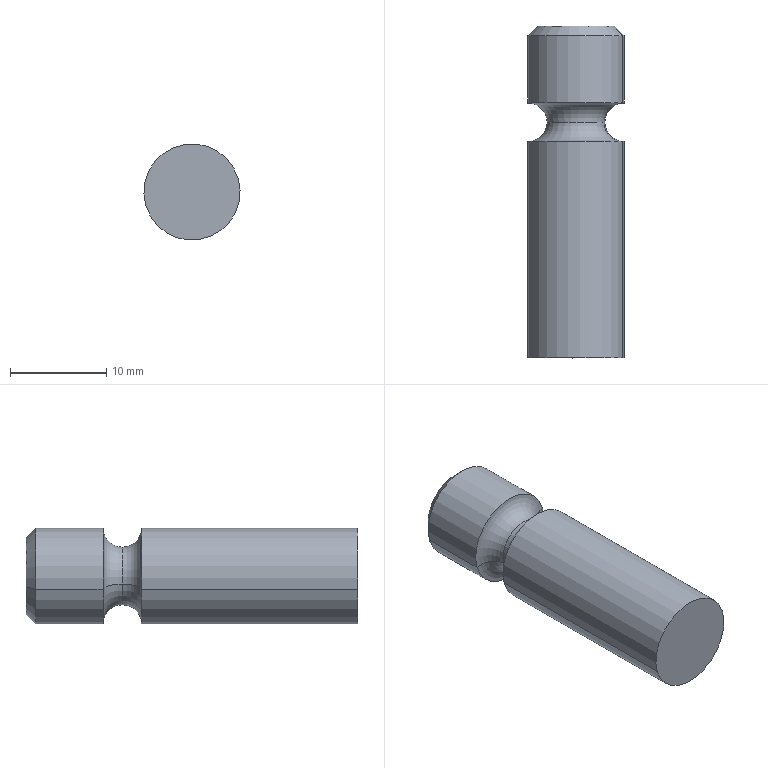Component | SolidWorks | 32-1 | 1 solid | 12 faces | box 10 x 34.5 x 10 mm | volume 2531 mm3 | torus 4 | cylinder 4 | cone 2 | plane 2 | commonest cylinder face diameters 10 x4
build123d program:
from build123d import *

# Parameters (mm, degrees)
SKETCH1_2_R             = 5
BOSS_EXTRUDE1_DEPTH     = 48
CHAMFER1_SIZE           = 1
CHAMFER2_SIZE           = 1
SKETCH3_R               = 2
CUT_EXTRUDE1_DEPTH      = 13.5
CUT_EXTRUDE1_DEPTH_BACK = 13.5
SKETCH1_R               = 6


with BuildPart() as part:
    # Sketch1_2 → Boss-Extrude1 (new body)
    with BuildSketch(Plane.XY):
        Circle(SKETCH1_2_R)
    extrude(amount=BOSS_EXTRUDE1_DEPTH)

    # Chamfer1
    chamfer1_edges = [part.edges().sort_by_distance(p)[0] for p in [
        (-5, 0, 0),
    ]]
    chamfer(chamfer1_edges, length=CHAMFER1_SIZE)

    # Chamfer2
    chamfer2_edges = [part.edges().sort_by_distance(p)[0] for p in [
        (-5, 0, 48),
    ]]
    chamfer(chamfer2_edges, length=CHAMFER2_SIZE)

    # Sketch3 → Cut-Revolve1 (revolve, cut)
    with BuildSketch(Plane(origin=(0, 0, 0), x_dir=(1, 0, 0), z_dir=(0, 1, 0))):
        with Locations((5, -38)):
            Circle(SKETCH3_R)
    revolve(axis=Axis((0, 0, 48), (0, 0, -1)), mode=Mode.SUBTRACT)

    # Sketch1 → Cut-Extrude1 (cut, two sides: drawn at the far end of the back side and taken through both)
    with BuildSketch(Plane.XY.offset(-CUT_EXTRUDE1_DEPTH_BACK)):
        Circle(SKETCH1_R)
    extrude(amount=CUT_EXTRUDE1_DEPTH + CUT_EXTRUDE1_DEPTH_BACK, mode=Mode.SUBTRACT)


solid = part.part

# Placed as in the assembly
solid = solid.moved(Location((17.957, 384.991, 382.093), (-90, 0, 0)))
STEP:
#1=CARTESIAN_POINT('',(0.518,16.732,14.988));
#2=VERTEX_POINT('',#1);
#3=CARTESIAN_POINT('',(0.5936,16.653,15.01));
#4=VERTEX_POINT('',#3);
#5=CARTESIAN_POINT('',(0.518,16.653,14.988));
#6=DIRECTION('',(0.2793,0.,-0.9602));
#7=DIRECTION('',(-0.9602,0.,-0.2793));
#8=AXIS2_PLACEMENT_3D('',#5,#6,#7);
#9=CIRCLE('',#8,0.07874);
#10=EDGE_CURVE('',#2,#4,#9,.T.);
#11=ORIENTED_EDGE('',*,*,#10,.T.);
#12=CARTESIAN_POINT('',(0.8204,16.653,15.076));
#13=VERTEX_POINT('',#12);
#14=CARTESIAN_POINT('',(0.707,16.653,15.043));
#15=DIRECTION('',(-0.,1.,0.));
#16=DIRECTION('',(-1.,0.,0.));
#17=AXIS2_PLACEMENT_3D('',#14,#15,#16);
#18=CIRCLE('',#17,0.1181);
#19=EDGE_CURVE('',#4,#13,#18,.T.);
#20=ORIENTED_EDGE('',*,*,#19,.T.);
#21=CARTESIAN_POINT('',(0.896,16.732,15.098));
#22=VERTEX_POINT('',#21);
#23=CARTESIAN_POINT('',(0.896,16.653,15.098));
#24=DIRECTION('',(-0.2793,-0.,0.9602));
#25=DIRECTION('',(0.9602,0.,0.2793));
#26=AXIS2_PLACEMENT_3D('',#23,#24,#25);
#27=CIRCLE('',#26,0.07874);
#28=EDGE_CURVE('',#22,#13,#27,.T.);
#29=ORIENTED_EDGE('',*,*,#28,.F.);
#30=CARTESIAN_POINT('',(0.707,16.732,15.043));
#31=DIRECTION('',(-0.,1.,0.));
#32=DIRECTION('',(0.9602,0.,0.2793));
#33=AXIS2_PLACEMENT_3D('',#30,#31,#32);
#34=CIRCLE('',#33,0.1969);
#35=EDGE_CURVE('',#2,#22,#34,.T.);
#36=ORIENTED_EDGE('',*,*,#35,.F.);
#37=EDGE_LOOP('',(#11,#20,#29,#36));
#38=FACE_OUTER_BOUND('',#37,.T.);
#39=CARTESIAN_POINT('',(0.707,16.653,15.043));
#40=DIRECTION('',(-0.,1.,0.));
#41=DIRECTION('',(-0.9602,-0.,-0.2793));
#42=AXIS2_PLACEMENT_3D('',#39,#40,#41);
#43=TOROIDAL_SURFACE('',#42,0.1969,0.07874);
#44=ADVANCED_FACE('',(#38),#43,.F.);
#45=ORIENTED_EDGE('',*,*,#28,.T.);
#46=CARTESIAN_POINT('',(0.707,16.653,15.043));
#47=DIRECTION('',(-0.,1.,0.));
#48=DIRECTION('',(-1.,0.,0.));
#49=AXIS2_PLACEMENT_3D('',#46,#47,#48);
#50=CIRCLE('',#49,0.1181);
#51=EDGE_CURVE('',#13,#4,#50,.T.);
#52=ORIENTED_EDGE('',*,*,#51,.T.);
#53=ORIENTED_EDGE('',*,*,#10,.F.);
#54=CARTESIAN_POINT('',(0.707,16.732,15.043));
#55=DIRECTION('',(-0.,1.,0.));
#56=DIRECTION('',(0.9602,0.,0.2793));
#57=AXIS2_PLACEMENT_3D('',#54,#55,#56);
#58=CIRCLE('',#57,0.1969);
#59=EDGE_CURVE('',#22,#2,#58,.T.);
#60=ORIENTED_EDGE('',*,*,#59,.F.);
#61=EDGE_LOOP('',(#45,#52,#53,#60));
#62=FACE_OUTER_BOUND('',#61,.T.);
#63=CARTESIAN_POINT('',(0.707,16.653,15.043));
#64=DIRECTION('',(-0.,1.,0.));
#65=DIRECTION('',(-0.9602,-0.,-0.2793));
#66=AXIS2_PLACEMENT_3D('',#63,#64,#65);
#67=TOROIDAL_SURFACE('',#66,0.1969,0.07874);
#68=ADVANCED_FACE('',(#62),#67,.F.);
#69=CARTESIAN_POINT('',(0.896,16.574,15.098));
#70=VERTEX_POINT('',#69);
#71=CARTESIAN_POINT('',(0.518,16.574,14.988));
#72=VERTEX_POINT('',#71);
#73=CARTESIAN_POINT('',(0.707,16.574,15.043));
#74=DIRECTION('',(0.,-1.,-0.));
#75=DIRECTION('',(-0.9602,0.,-0.2793));
#76=AXIS2_PLACEMENT_3D('',#73,#74,#75);
#77=CIRCLE('',#76,0.1969);
#78=EDGE_CURVE('',#70,#72,#77,.T.);
#79=ORIENTED_EDGE('',*,*,#78,.T.);
#80=CARTESIAN_POINT('',(0.518,15.689,14.988));
#81=VERTEX_POINT('',#80);
#82=CARTESIAN_POINT('',(0.518,17.047,14.988));
#83=DIRECTION('',(0.,-1.,-0.));
#84=VECTOR('',#83,39.37);
#85=LINE('',#82,#84);
#86=EDGE_CURVE('',#72,#81,#85,.T.);
#87=ORIENTED_EDGE('',*,*,#86,.T.);
#88=CARTESIAN_POINT('',(0.896,15.689,15.098));
#89=VERTEX_POINT('',#88);
#90=CARTESIAN_POINT('',(0.707,15.689,15.043));
#91=DIRECTION('',(-0.,1.,0.));
#92=DIRECTION('',(-0.9602,0.,-0.2793));
#93=AXIS2_PLACEMENT_3D('',#90,#91,#92);
#94=CIRCLE('',#93,0.1969);
#95=EDGE_CURVE('',#81,#89,#94,.T.);
#96=ORIENTED_EDGE('',*,*,#95,.T.);
#97=CARTESIAN_POINT('',(0.896,17.047,15.098));
#98=DIRECTION('',(0.,-1.,-0.));
#99=VECTOR('',#98,39.37);
#100=LINE('',#97,#99);
#101=EDGE_CURVE('',#70,#89,#100,.T.);
#102=ORIENTED_EDGE('',*,*,#101,.F.);
#103=EDGE_LOOP('',(#79,#87,#96,#102));
#104=FACE_OUTER_BOUND('',#103,.T.);
#105=CARTESIAN_POINT('',(0.707,17.047,15.043));
#106=DIRECTION('',(0.,-1.,-0.));
#107=DIRECTION('',(0.9602,0.,0.2793));
#108=AXIS2_PLACEMENT_3D('',#105,#106,#107);
#109=CYLINDRICAL_SURFACE('',#108,0.1969);
#110=ADVANCED_FACE('',(#104),#109,.T.);
#111=ORIENTED_EDGE('',*,*,#51,.F.);
#112=CARTESIAN_POINT('',(0.896,16.653,15.098));
#113=DIRECTION('',(-0.2793,-0.,0.9602));
#114=DIRECTION('',(0.9602,0.,0.2793));
#115=AXIS2_PLACEMENT_3D('',#112,#113,#114);
#116=CIRCLE('',#115,0.07874);
#117=EDGE_CURVE('',#13,#70,#116,.T.);
#118=ORIENTED_EDGE('',*,*,#117,.T.);
#119=CARTESIAN_POINT('',(0.707,16.574,15.043));
#120=DIRECTION('',(0.,-1.,-0.));
#121=DIRECTION('',(-0.9602,0.,-0.2793));
#122=AXIS2_PLACEMENT_3D('',#119,#120,#121);
#123=CIRCLE('',#122,0.1969);
#124=EDGE_CURVE('',#72,#70,#123,.T.);
#125=ORIENTED_EDGE('',*,*,#124,.F.);
#126=CARTESIAN_POINT('',(0.518,16.653,14.988));
#127=DIRECTION('',(0.2793,0.,-0.9602));
#128=DIRECTION('',(-0.9602,0.,-0.2793));
#129=AXIS2_PLACEMENT_3D('',#126,#127,#128);
#130=CIRCLE('',#129,0.07874);
#131=EDGE_CURVE('',#4,#72,#130,.T.);
#132=ORIENTED_EDGE('',*,*,#131,.F.);
#133=EDGE_LOOP('',(#111,#118,#125,#132));
#134=FACE_OUTER_BOUND('',#133,.T.);
#135=CARTESIAN_POINT('',(0.707,16.653,15.043));
#136=DIRECTION('',(-0.,1.,0.));
#137=DIRECTION('',(-0.9602,-0.,-0.2793));
#138=AXIS2_PLACEMENT_3D('',#135,#136,#137);
#139=TOROIDAL_SURFACE('',#138,0.1969,0.07874);
#140=ADVANCED_FACE('',(#134),#139,.F.);
#141=CARTESIAN_POINT('',(0.5558,17.047,14.999));
#142=VERTEX_POINT('',#141);
#143=CARTESIAN_POINT('',(0.8582,17.047,15.087));
#144=VERTEX_POINT('',#143);
#145=CARTESIAN_POINT('',(0.707,17.047,15.043));
#146=DIRECTION('',(-0.,1.,0.));
#147=DIRECTION('',(-0.9602,0.,-0.2793));
#148=AXIS2_PLACEMENT_3D('',#145,#146,#147);
#149=CIRCLE('',#148,0.1575);
#150=EDGE_CURVE('',#142,#144,#149,.T.);
#151=ORIENTED_EDGE('',*,*,#150,.F.);
#152=CARTESIAN_POINT('',(0.518,17.008,14.988));
#153=VERTEX_POINT('',#152);
#154=CARTESIAN_POINT('',(0.5558,17.047,14.999));
#155=DIRECTION('',(-0.679,-0.7071,-0.1975));
#156=VECTOR('',#155,39.37);
#157=LINE('',#154,#156);
#158=EDGE_CURVE('',#142,#153,#157,.T.);
#159=ORIENTED_EDGE('',*,*,#158,.T.);
#160=CARTESIAN_POINT('',(0.896,17.008,15.098));
#161=VERTEX_POINT('',#160);
#162=CARTESIAN_POINT('',(0.707,17.008,15.043));
#163=DIRECTION('',(0.,-1.,-0.));
#164=DIRECTION('',(-0.9602,0.,-0.2793));
#165=AXIS2_PLACEMENT_3D('',#162,#163,#164);
#166=CIRCLE('',#165,0.1969);
#167=EDGE_CURVE('',#161,#153,#166,.T.);
#168=ORIENTED_EDGE('',*,*,#167,.F.);
#169=CARTESIAN_POINT('',(0.8582,17.047,15.087));
#170=DIRECTION('',(0.679,-0.7071,0.1975));
#171=VECTOR('',#170,39.37);
#172=LINE('',#169,#171);
#173=EDGE_CURVE('',#144,#161,#172,.T.);
#174=ORIENTED_EDGE('',*,*,#173,.F.);
#175=EDGE_LOOP('',(#151,#159,#168,#174));
#176=FACE_OUTER_BOUND('',#175,.T.);
#177=CARTESIAN_POINT('',(0.707,17.047,15.043));
#178=DIRECTION('',(0.,-1.,-0.));
#179=DIRECTION('',(0.9602,0.,0.2793));
#180=AXIS2_PLACEMENT_3D('',#177,#178,#179);
#181=CONICAL_SURFACE('',#180,0.1575,0.7854);
#182=ADVANCED_FACE('',(#176),#181,.T.);
#183=ORIENTED_EDGE('',*,*,#167,.T.);
#184=CARTESIAN_POINT('',(0.518,17.047,14.988));
#185=DIRECTION('',(0.,-1.,-0.));
#186=VECTOR('',#185,39.37);
#187=LINE('',#184,#186);
#188=EDGE_CURVE('',#153,#2,#187,.T.);
#189=ORIENTED_EDGE('',*,*,#188,.T.);
#190=ORIENTED_EDGE('',*,*,#35,.T.);
#191=CARTESIAN_POINT('',(0.896,17.047,15.098));
#192=DIRECTION('',(0.,-1.,-0.));
#193=VECTOR('',#192,39.37);
#194=LINE('',#191,#193);
#195=EDGE_CURVE('',#161,#22,#194,.T.);
#196=ORIENTED_EDGE('',*,*,#195,.F.);
#197=EDGE_LOOP('',(#183,#189,#190,#196));
#198=FACE_OUTER_BOUND('',#197,.T.);
#199=CARTESIAN_POINT('',(0.707,17.047,15.043));
#200=DIRECTION('',(0.,-1.,-0.));
#201=DIRECTION('',(0.9602,0.,0.2793));
#202=AXIS2_PLACEMENT_3D('',#199,#200,#201);
#203=CYLINDRICAL_SURFACE('',#202,0.1969);
#204=ADVANCED_FACE('',(#198),#203,.T.);
#205=ORIENTED_EDGE('',*,*,#188,.F.);
#206=CARTESIAN_POINT('',(0.707,17.008,15.043));
#207=DIRECTION('',(0.,-1.,-0.));
#208=DIRECTION('',(-0.9602,0.,-0.2793));
#209=AXIS2_PLACEMENT_3D('',#206,#207,#208);
#210=CIRCLE('',#209,0.1969);
#211=EDGE_CURVE('',#153,#161,#210,.T.);
#212=ORIENTED_EDGE('',*,*,#211,.T.);
#213=ORIENTED_EDGE('',*,*,#195,.T.);
#214=ORIENTED_EDGE('',*,*,#59,.T.);
#215=EDGE_LOOP('',(#205,#212,#213,#214));
#216=FACE_OUTER_BOUND('',#215,.T.);
#217=CARTESIAN_POINT('',(0.707,17.047,15.043));
#218=DIRECTION('',(0.,-1.,-0.));
#219=DIRECTION('',(0.9602,0.,0.2793));
#220=AXIS2_PLACEMENT_3D('',#217,#218,#219);
#221=CYLINDRICAL_SURFACE('',#220,0.1969);
#222=ADVANCED_FACE('',(#216),#221,.T.);
#223=CARTESIAN_POINT('',(0.707,17.047,15.043));
#224=DIRECTION('',(-0.,1.,0.));
#225=DIRECTION('',(-0.9602,0.,-0.2793));
#226=AXIS2_PLACEMENT_3D('',#223,#224,#225);
#227=CIRCLE('',#226,0.1575);
#228=EDGE_CURVE('',#144,#142,#227,.T.);
#229=ORIENTED_EDGE('',*,*,#228,.T.);
#230=ORIENTED_EDGE('',*,*,#150,.T.);
#231=EDGE_LOOP('',(#229,#230));
#232=FACE_OUTER_BOUND('',#231,.T.);
#233=CARTESIAN_POINT('',(0.707,17.047,15.043));
#234=DIRECTION('',(-0.,1.,0.));
#235=DIRECTION('',(-0.9602,-0.,-0.2793));
#236=AXIS2_PLACEMENT_3D('',#233,#234,#235);
#237=PLANE('',#236);
#238=ADVANCED_FACE('',(#232),#237,.T.);
#239=ORIENTED_EDGE('',*,*,#158,.F.);
#240=ORIENTED_EDGE('',*,*,#228,.F.);
#241=ORIENTED_EDGE('',*,*,#173,.T.);
#242=ORIENTED_EDGE('',*,*,#211,.F.);
#243=EDGE_LOOP('',(#239,#240,#241,#242));
#244=FACE_OUTER_BOUND('',#243,.T.);
#245=CARTESIAN_POINT('',(0.707,17.047,15.043));
#246=DIRECTION('',(0.,-1.,-0.));
#247=DIRECTION('',(0.9602,0.,0.2793));
#248=AXIS2_PLACEMENT_3D('',#245,#246,#247);
#249=CONICAL_SURFACE('',#248,0.1575,0.7854);
#250=ADVANCED_FACE('',(#244),#249,.T.);
#251=ORIENTED_EDGE('',*,*,#19,.F.);
#252=ORIENTED_EDGE('',*,*,#131,.T.);
#253=ORIENTED_EDGE('',*,*,#78,.F.);
#254=ORIENTED_EDGE('',*,*,#117,.F.);
#255=EDGE_LOOP('',(#251,#252,#253,#254));
#256=FACE_OUTER_BOUND('',#255,.T.);
#257=CARTESIAN_POINT('',(0.707,16.653,15.043));
#258=DIRECTION('',(-0.,1.,0.));
#259=DIRECTION('',(-0.9602,-0.,-0.2793));
#260=AXIS2_PLACEMENT_3D('',#257,#258,#259);
#261=TOROIDAL_SURFACE('',#260,0.1969,0.07874);
#262=ADVANCED_FACE('',(#256),#261,.F.);
#263=ORIENTED_EDGE('',*,*,#86,.F.);
#264=ORIENTED_EDGE('',*,*,#124,.T.);
#265=ORIENTED_EDGE('',*,*,#101,.T.);
#266=CARTESIAN_POINT('',(0.707,15.689,15.043));
#267=DIRECTION('',(-0.,1.,0.));
#268=DIRECTION('',(-0.9602,0.,-0.2793));
#269=AXIS2_PLACEMENT_3D('',#266,#267,#268);
#270=CIRCLE('',#269,0.1969);
#271=EDGE_CURVE('',#89,#81,#270,.T.);
#272=ORIENTED_EDGE('',*,*,#271,.T.);
#273=EDGE_LOOP('',(#263,#264,#265,#272));
#274=FACE_OUTER_BOUND('',#273,.T.);
#275=CARTESIAN_POINT('',(0.707,17.047,15.043));
#276=DIRECTION('',(0.,-1.,-0.));
#277=DIRECTION('',(0.9602,0.,0.2793));
#278=AXIS2_PLACEMENT_3D('',#275,#276,#277);
#279=CYLINDRICAL_SURFACE('',#278,0.1969);
#280=ADVANCED_FACE('',(#274),#279,.T.);
#281=ORIENTED_EDGE('',*,*,#271,.F.);
#282=ORIENTED_EDGE('',*,*,#95,.F.);
#283=EDGE_LOOP('',(#281,#282));
#284=FACE_OUTER_BOUND('',#283,.T.);
#285=CARTESIAN_POINT('',(0.707,15.689,15.043));
#286=DIRECTION('',(-0.,1.,0.));
#287=DIRECTION('',(-0.9602,-0.,-0.2793));
#288=AXIS2_PLACEMENT_3D('',#285,#286,#287);
#289=PLANE('',#288);
#290=ADVANCED_FACE('',(#284),#289,.F.);
#291=CLOSED_SHELL('',(#44,#68,#110,#140,#182,#204,#222,#238,#250,#262,#280,#290));
#292=MANIFOLD_SOLID_BREP('',#291);
#293=CARTESIAN_POINT('',(0.,0.,0.));
#294=DIRECTION('',(0.,0.,1.));
#295=DIRECTION('',(1.,0.,0.));
#296=AXIS2_PLACEMENT_3D('',#293,#294,#295);
#297=(LENGTH_UNIT()NAMED_UNIT(*)SI_UNIT($,.METRE.));
#298=LENGTH_MEASURE_WITH_UNIT(LENGTH_MEASURE(0.0254),#297);
#299=DIMENSIONAL_EXPONENTS(1.,0.,0.,0.,0.,0.,0.);
#300=(CONVERSION_BASED_UNIT('',#298)LENGTH_UNIT()NAMED_UNIT(#299));
#301=UNCERTAINTY_MEASURE_WITH_UNIT(LENGTH_MEASURE(0.00001),#300,'','');
#302=(NAMED_UNIT(*)PLANE_ANGLE_UNIT()SI_UNIT($,.RADIAN.));
#303=(NAMED_UNIT(*)SI_UNIT($,.STERADIAN.)SOLID_ANGLE_UNIT());
#304=(GEOMETRIC_REPRESENTATION_CONTEXT(3)GLOBAL_UNCERTAINTY_ASSIGNED_CONTEXT((#301))GLOBAL_UNIT_ASSIGNED_CONTEXT((#300,#302,#303))REPRESENTATION_CONTEXT('',''));
#305=ADVANCED_BREP_SHAPE_REPRESENTATION('',(#292,#296),#304);
#306=COLOUR_RGB('',0.7922,0.8196,0.9333);
#307=FILL_AREA_STYLE_COLOUR('',#306);
#308=FILL_AREA_STYLE('',(#307));
#309=SURFACE_STYLE_FILL_AREA(#308);
#310=SURFACE_SIDE_STYLE('',(#309));
#311=SURFACE_STYLE_USAGE(.BOTH.,#310);
#312=PRESENTATION_STYLE_ASSIGNMENT((#311));
#313=STYLED_ITEM('',(#312),#292);
#314=PRESENTATION_LAYER_ASSIGNMENT('','',(#313));
#315=(LENGTH_UNIT()NAMED_UNIT(*)SI_UNIT($,.METRE.));
#316=LENGTH_MEASURE_WITH_UNIT(LENGTH_MEASURE(0.0254),#315);
#317=DIMENSIONAL_EXPONENTS(1.,0.,0.,0.,0.,0.,0.);
#318=(CONVERSION_BASED_UNIT('',#316)LENGTH_UNIT()NAMED_UNIT(#317));
#319=UNCERTAINTY_MEASURE_WITH_UNIT(LENGTH_MEASURE(0.00001),#318,'','');
#320=(NAMED_UNIT(*)PLANE_ANGLE_UNIT()SI_UNIT($,.RADIAN.));
#321=(NAMED_UNIT(*)SI_UNIT($,.STERADIAN.)SOLID_ANGLE_UNIT());
#322=(GEOMETRIC_REPRESENTATION_CONTEXT(3)GLOBAL_UNCERTAINTY_ASSIGNED_CONTEXT((#319))GLOBAL_UNIT_ASSIGNED_CONTEXT((#318,#320,#321))REPRESENTATION_CONTEXT('',''));
#323=MECHANICAL_DESIGN_GEOMETRIC_PRESENTATION_REPRESENTATION('',(#313),#322);